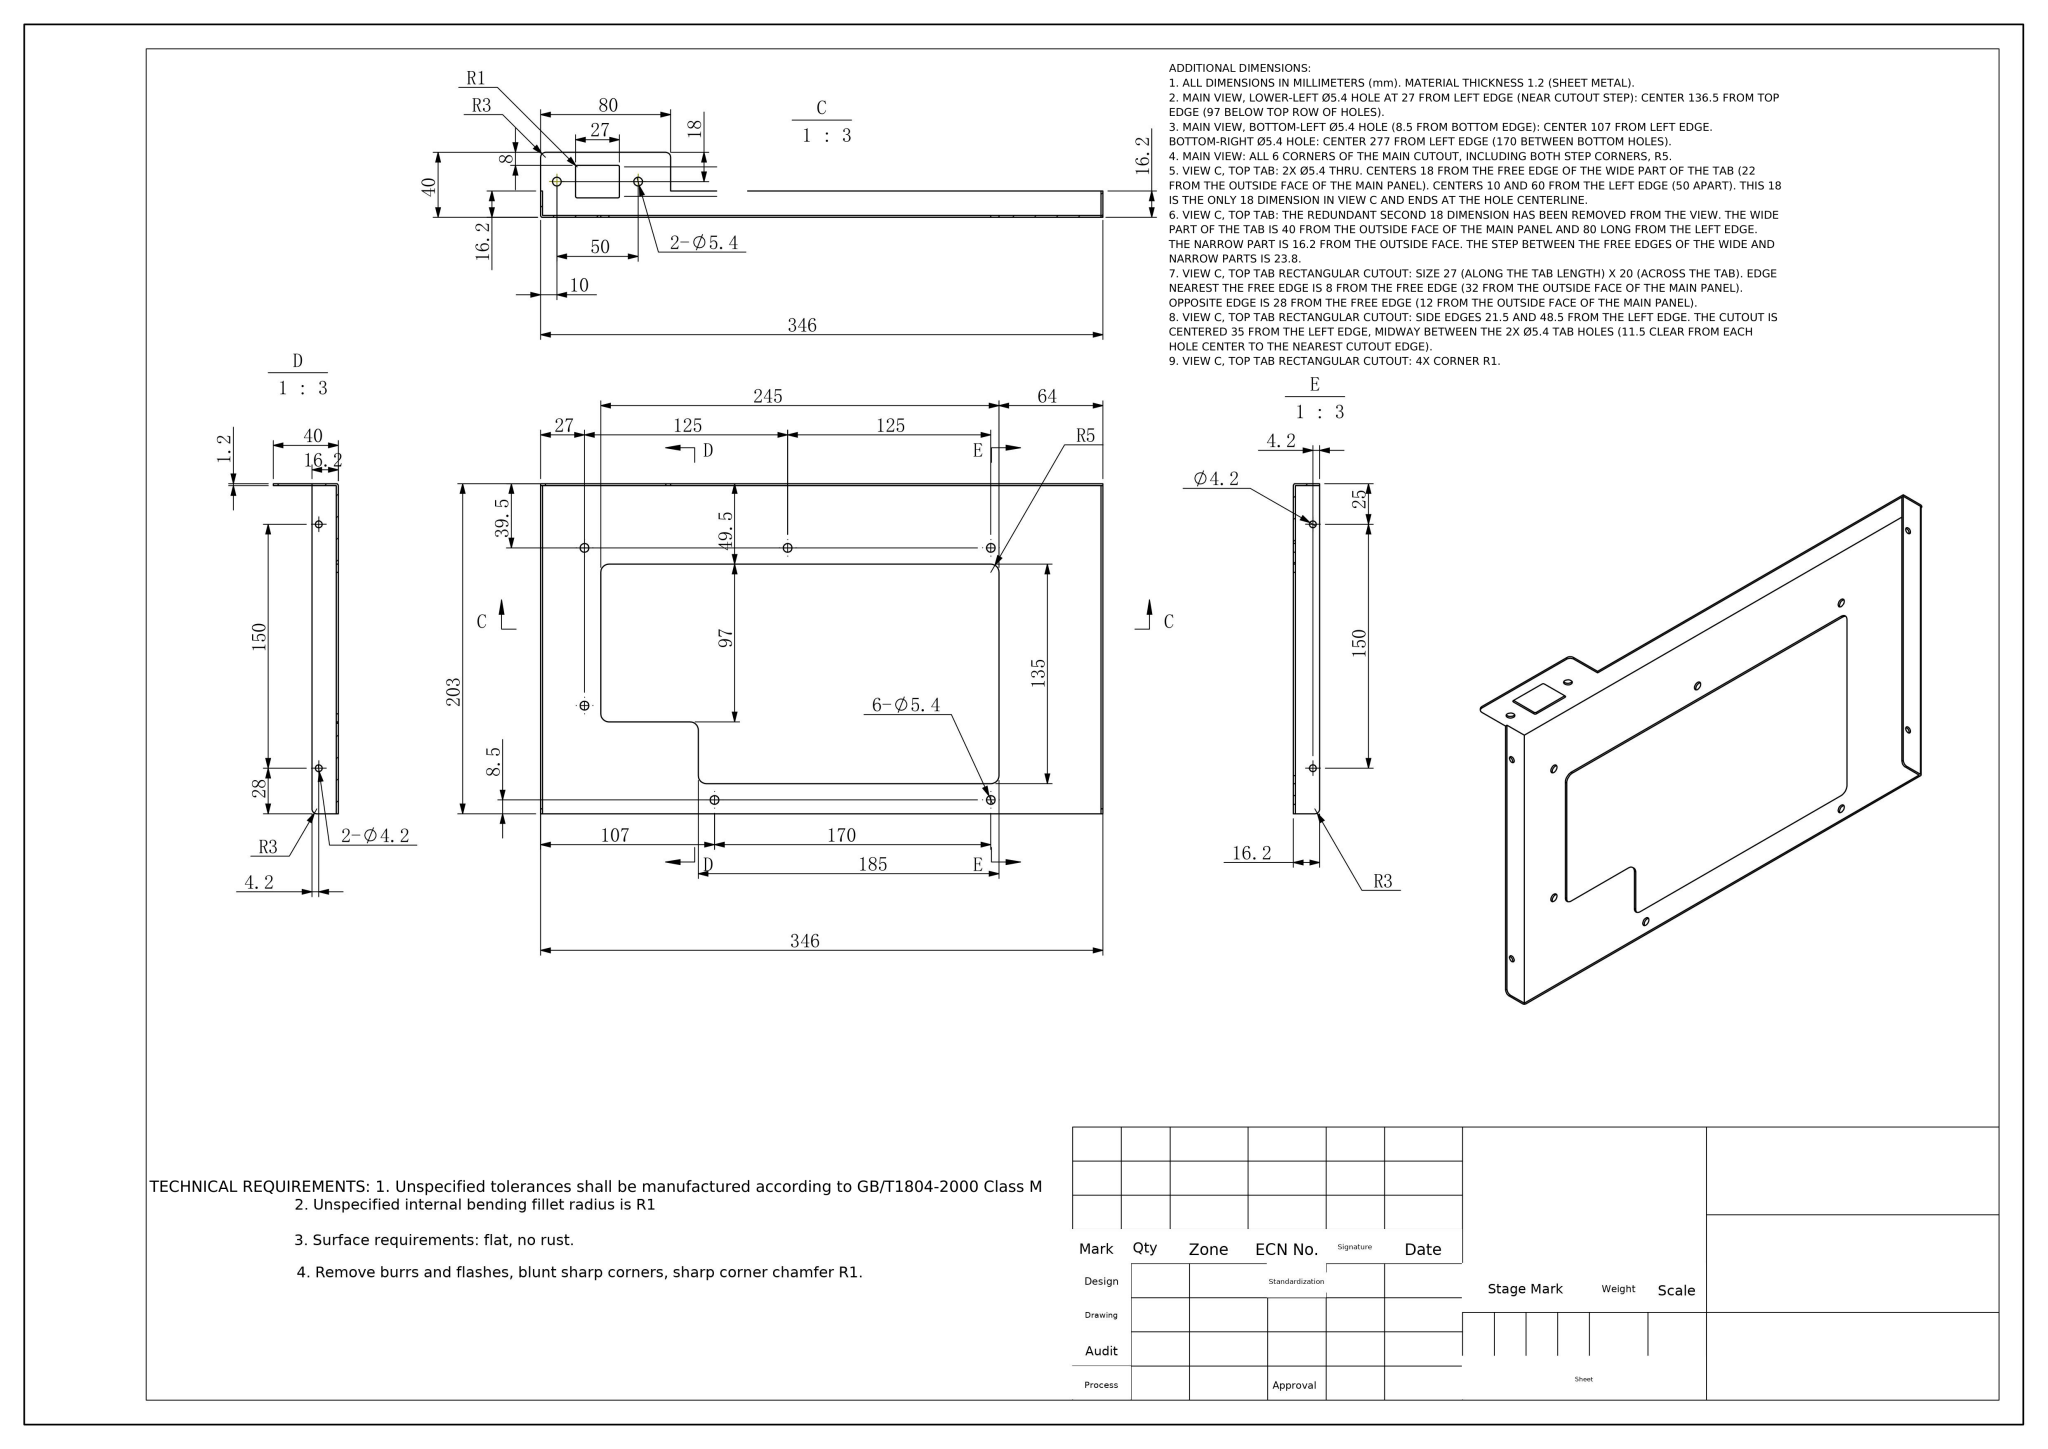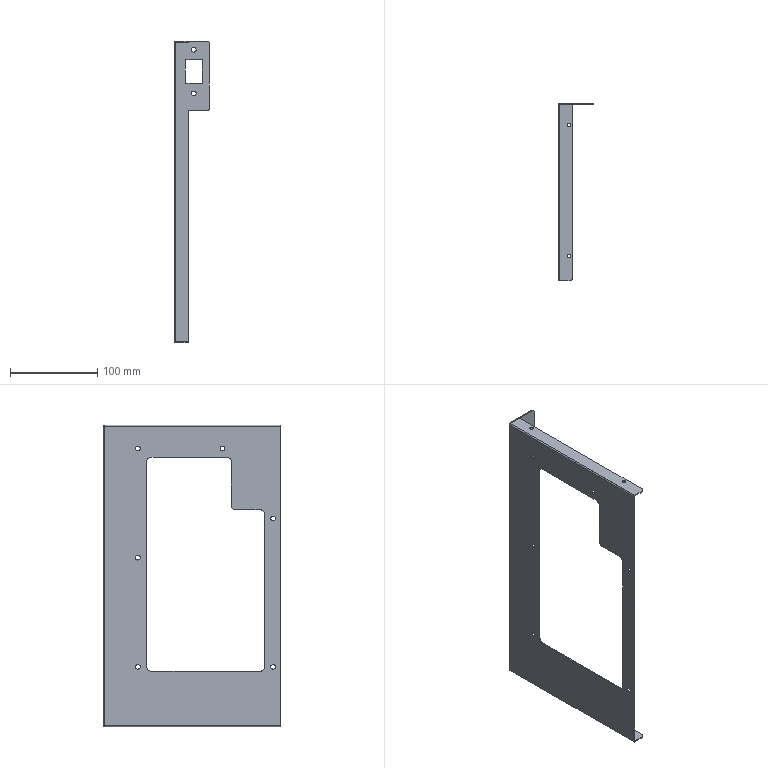Part | NX | mm | 1 solid | 76 faces | box 40 x 203 x 346 mm | volume 61958 mm3 | cylinder 44 | plane 32 | commonest cylinder face diameters 5.4 x16 4.2 x8 10 x6 2 x4 6 x4 2.404 x3 0.004 x3